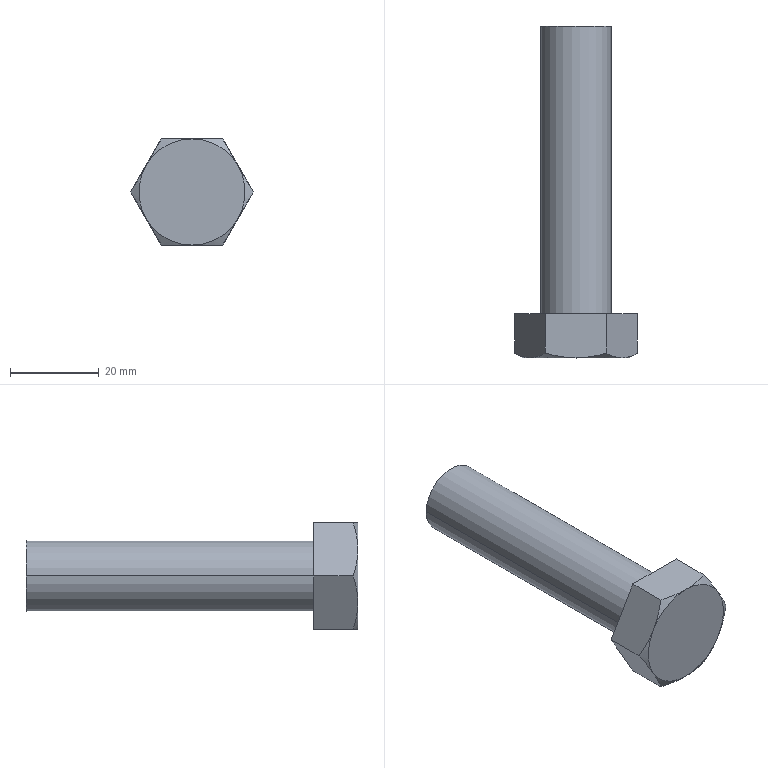Component | SolidWorks | Screw-1 | 1 solid | 17 faces | box 27.71 x 75 x 24 mm | volume 18042 mm3 | plane 9 | cone 6 | cylinder 2 | commonest cylinder face diameters 16 x2
STEP:
#1=COLOUR_RGB('',0.7922,0.8196,0.9333);
#2=FILL_AREA_STYLE_COLOUR('',#1);
#3=FILL_AREA_STYLE('',(#2));
#4=SURFACE_STYLE_FILL_AREA(#3);
#5=SURFACE_SIDE_STYLE('',(#4));
#6=SURFACE_STYLE_USAGE(.BOTH.,#5);
#7=PRESENTATION_STYLE_ASSIGNMENT((#6));
#8=CARTESIAN_POINT('',(-26.588,35.927,34.002));
#9=VERTEX_POINT('',#8);
#10=CARTESIAN_POINT('',(-25.958,35.927,34.002));
#11=VERTEX_POINT('',#10);
#12=CARTESIAN_POINT('',(-26.273,35.927,34.002));
#13=DIRECTION('',(0.,1.,0.));
#14=DIRECTION('',(-1.,0.,0.));
#15=AXIS2_PLACEMENT_3D('',#12,#13,#14);
#16=CIRCLE('',#15,0.315);
#17=EDGE_CURVE('',#9,#11,#16,.T.);
#18=ORIENTED_EDGE('',*,*,#17,.T.);
#19=CARTESIAN_POINT('',(-25.958,38.486,34.002));
#20=VERTEX_POINT('',#19);
#21=CARTESIAN_POINT('',(-25.958,35.927,34.002));
#22=DIRECTION('',(0.,1.,0.));
#23=VECTOR('',#22,39.37);
#24=LINE('',#21,#23);
#25=EDGE_CURVE('',#11,#20,#24,.T.);
#26=ORIENTED_EDGE('',*,*,#25,.T.);
#27=CARTESIAN_POINT('',(-26.588,38.486,34.002));
#28=VERTEX_POINT('',#27);
#29=CARTESIAN_POINT('',(-26.273,38.486,34.002));
#30=DIRECTION('',(0.,1.,0.));
#31=DIRECTION('',(-1.,0.,0.));
#32=AXIS2_PLACEMENT_3D('',#29,#30,#31);
#33=CIRCLE('',#32,0.315);
#34=EDGE_CURVE('',#28,#20,#33,.T.);
#35=ORIENTED_EDGE('',*,*,#34,.F.);
#36=CARTESIAN_POINT('',(-26.588,35.927,34.002));
#37=DIRECTION('',(0.,1.,0.));
#38=VECTOR('',#37,39.37);
#39=LINE('',#36,#38);
#40=EDGE_CURVE('',#9,#28,#39,.T.);
#41=ORIENTED_EDGE('',*,*,#40,.F.);
#42=EDGE_LOOP('',(#18,#26,#35,#41));
#43=FACE_OUTER_BOUND('',#42,.T.);
#44=CARTESIAN_POINT('',(-26.273,35.927,34.002));
#45=DIRECTION('',(0.,1.,0.));
#46=DIRECTION('',(-1.,0.,0.));
#47=AXIS2_PLACEMENT_3D('',#44,#45,#46);
#48=CYLINDRICAL_SURFACE('',#47,0.315);
#49=ADVANCED_FACE('',(#43),#48,.T.);
#50=CARTESIAN_POINT('',(-26.546,35.576,33.53));
#51=VERTEX_POINT('',#50);
#52=CARTESIAN_POINT('',(-26.273,35.533,33.53));
#53=VERTEX_POINT('',#52);
#54=CARTESIAN_POINT('',(-26.546,35.576,33.53));
#55=CARTESIAN_POINT('',(-26.501,35.563,33.53));
#56=CARTESIAN_POINT('',(-26.456,35.552,33.53));
#57=CARTESIAN_POINT('',(-26.365,35.537,33.53));
#58=CARTESIAN_POINT('',(-26.319,35.533,33.53));
#59=CARTESIAN_POINT('',(-26.273,35.533,33.53));
#60=B_SPLINE_CURVE_WITH_KNOTS('',3,(#54,#55,#56,#57,#58,#59),.UNSPECIFIED.,.F.,.F.,(4,2,4),(0.,0.003505,0.007011),.UNSPECIFIED.);
#61=EDGE_CURVE('',#51,#53,#60,.T.);
#62=ORIENTED_EDGE('',*,*,#61,.F.);
#63=CARTESIAN_POINT('',(-26.546,35.927,33.53));
#64=VERTEX_POINT('',#63);
#65=CARTESIAN_POINT('',(-26.546,35.927,33.53));
#66=DIRECTION('',(0.,-1.,0.));
#67=VECTOR('',#66,39.37);
#68=LINE('',#65,#67);
#69=EDGE_CURVE('',#64,#51,#68,.T.);
#70=ORIENTED_EDGE('',*,*,#69,.F.);
#71=CARTESIAN_POINT('',(-26.,35.927,33.53));
#72=VERTEX_POINT('',#71);
#73=CARTESIAN_POINT('',(-26.546,35.927,33.53));
#74=DIRECTION('',(-1.,0.,0.));
#75=VECTOR('',#74,39.37);
#76=LINE('',#73,#75);
#77=EDGE_CURVE('',#72,#64,#76,.T.);
#78=ORIENTED_EDGE('',*,*,#77,.F.);
#79=CARTESIAN_POINT('',(-26.,35.576,33.53));
#80=VERTEX_POINT('',#79);
#81=CARTESIAN_POINT('',(-26.,35.927,33.53));
#82=DIRECTION('',(0.,-1.,0.));
#83=VECTOR('',#82,39.37);
#84=LINE('',#81,#83);
#85=EDGE_CURVE('',#72,#80,#84,.T.);
#86=ORIENTED_EDGE('',*,*,#85,.T.);
#87=CARTESIAN_POINT('',(-26.273,35.533,33.53));
#88=CARTESIAN_POINT('',(-26.226,35.533,33.53));
#89=CARTESIAN_POINT('',(-26.18,35.537,33.53));
#90=CARTESIAN_POINT('',(-26.09,35.552,33.53));
#91=CARTESIAN_POINT('',(-26.045,35.563,33.53));
#92=CARTESIAN_POINT('',(-26.,35.576,33.53));
#93=B_SPLINE_CURVE_WITH_KNOTS('',3,(#87,#88,#89,#90,#91,#92),.UNSPECIFIED.,.F.,.F.,(4,2,4),(0.,0.003505,0.007011),.UNSPECIFIED.);
#94=EDGE_CURVE('',#53,#80,#93,.T.);
#95=ORIENTED_EDGE('',*,*,#94,.F.);
#96=EDGE_LOOP('',(#62,#70,#78,#86,#95));
#97=FACE_OUTER_BOUND('',#96,.T.);
#98=CARTESIAN_POINT('',(-26.,35.533,33.53));
#99=DIRECTION('',(0.,0.,1.));
#100=DIRECTION('',(1.,0.,0.));
#101=AXIS2_PLACEMENT_3D('',#98,#99,#100);
#102=PLANE('',#101);
#103=ADVANCED_FACE('',(#97),#102,.F.);
#104=CARTESIAN_POINT('',(-26.818,35.576,34.002));
#105=VERTEX_POINT('',#104);
#106=CARTESIAN_POINT('',(-26.682,35.533,33.766));
#107=VERTEX_POINT('',#106);
#108=CARTESIAN_POINT('',(-26.818,35.576,34.002));
#109=CARTESIAN_POINT('',(-26.796,35.563,33.964));
#110=CARTESIAN_POINT('',(-26.774,35.552,33.925));
#111=CARTESIAN_POINT('',(-26.728,35.537,33.846));
#112=CARTESIAN_POINT('',(-26.705,35.533,33.807));
#113=CARTESIAN_POINT('',(-26.682,35.533,33.766));
#114=B_SPLINE_CURVE_WITH_KNOTS('',3,(#108,#109,#110,#111,#112,#113),.UNSPECIFIED.,.F.,.F.,(4,2,4),(0.,0.003505,0.007011),.UNSPECIFIED.);
#115=EDGE_CURVE('',#105,#107,#114,.T.);
#116=ORIENTED_EDGE('',*,*,#115,.F.);
#117=CARTESIAN_POINT('',(-26.818,35.927,34.002));
#118=VERTEX_POINT('',#117);
#119=CARTESIAN_POINT('',(-26.818,35.927,34.002));
#120=DIRECTION('',(0.,-1.,0.));
#121=VECTOR('',#120,39.37);
#122=LINE('',#119,#121);
#123=EDGE_CURVE('',#118,#105,#122,.T.);
#124=ORIENTED_EDGE('',*,*,#123,.F.);
#125=CARTESIAN_POINT('',(-26.818,35.927,34.002));
#126=DIRECTION('',(-0.5,0.,0.866));
#127=VECTOR('',#126,39.37);
#128=LINE('',#125,#127);
#129=EDGE_CURVE('',#64,#118,#128,.T.);
#130=ORIENTED_EDGE('',*,*,#129,.F.);
#131=ORIENTED_EDGE('',*,*,#69,.T.);
#132=CARTESIAN_POINT('',(-26.682,35.533,33.766));
#133=CARTESIAN_POINT('',(-26.659,35.533,33.726));
#134=CARTESIAN_POINT('',(-26.636,35.537,33.686));
#135=CARTESIAN_POINT('',(-26.59,35.552,33.608));
#136=CARTESIAN_POINT('',(-26.568,35.563,33.569));
#137=CARTESIAN_POINT('',(-26.546,35.576,33.53));
#138=B_SPLINE_CURVE_WITH_KNOTS('',3,(#132,#133,#134,#135,#136,#137),.UNSPECIFIED.,.F.,.F.,(4,2,4),(0.,0.003505,0.007011),.UNSPECIFIED.);
#139=EDGE_CURVE('',#107,#51,#138,.T.);
#140=ORIENTED_EDGE('',*,*,#139,.F.);
#141=EDGE_LOOP('',(#116,#124,#130,#131,#140));
#142=FACE_OUTER_BOUND('',#141,.T.);
#143=CARTESIAN_POINT('',(-26.546,35.533,33.53));
#144=DIRECTION('',(0.866,0.,0.5));
#145=DIRECTION('',(0.5,0.,-0.866));
#146=AXIS2_PLACEMENT_3D('',#143,#144,#145);
#147=PLANE('',#146);
#148=ADVANCED_FACE('',(#142),#147,.F.);
#149=CARTESIAN_POINT('',(-26.546,35.576,34.475));
#150=VERTEX_POINT('',#149);
#151=CARTESIAN_POINT('',(-26.682,35.533,34.239));
#152=VERTEX_POINT('',#151);
#153=CARTESIAN_POINT('',(-26.546,35.576,34.475));
#154=CARTESIAN_POINT('',(-26.568,35.563,34.436));
#155=CARTESIAN_POINT('',(-26.59,35.552,34.397));
#156=CARTESIAN_POINT('',(-26.636,35.537,34.319));
#157=CARTESIAN_POINT('',(-26.659,35.533,34.279));
#158=CARTESIAN_POINT('',(-26.682,35.533,34.239));
#159=B_SPLINE_CURVE_WITH_KNOTS('',3,(#153,#154,#155,#156,#157,#158),.UNSPECIFIED.,.F.,.F.,(4,2,4),(0.,0.003505,0.007011),.UNSPECIFIED.);
#160=EDGE_CURVE('',#150,#152,#159,.T.);
#161=ORIENTED_EDGE('',*,*,#160,.F.);
#162=CARTESIAN_POINT('',(-26.546,35.927,34.475));
#163=VERTEX_POINT('',#162);
#164=CARTESIAN_POINT('',(-26.546,35.927,34.475));
#165=DIRECTION('',(0.,-1.,0.));
#166=VECTOR('',#165,39.37);
#167=LINE('',#164,#166);
#168=EDGE_CURVE('',#163,#150,#167,.T.);
#169=ORIENTED_EDGE('',*,*,#168,.F.);
#170=CARTESIAN_POINT('',(-26.546,35.927,34.475));
#171=DIRECTION('',(0.5,0.,0.866));
#172=VECTOR('',#171,39.37);
#173=LINE('',#170,#172);
#174=EDGE_CURVE('',#118,#163,#173,.T.);
#175=ORIENTED_EDGE('',*,*,#174,.F.);
#176=ORIENTED_EDGE('',*,*,#123,.T.);
#177=CARTESIAN_POINT('',(-26.682,35.533,34.239));
#178=CARTESIAN_POINT('',(-26.705,35.533,34.198));
#179=CARTESIAN_POINT('',(-26.728,35.537,34.159));
#180=CARTESIAN_POINT('',(-26.774,35.552,34.08));
#181=CARTESIAN_POINT('',(-26.796,35.563,34.041));
#182=CARTESIAN_POINT('',(-26.818,35.576,34.002));
#183=B_SPLINE_CURVE_WITH_KNOTS('',3,(#177,#178,#179,#180,#181,#182),.UNSPECIFIED.,.F.,.F.,(4,2,4),(0.,0.003505,0.007011),.UNSPECIFIED.);
#184=EDGE_CURVE('',#152,#105,#183,.T.);
#185=ORIENTED_EDGE('',*,*,#184,.F.);
#186=EDGE_LOOP('',(#161,#169,#175,#176,#185));
#187=FACE_OUTER_BOUND('',#186,.T.);
#188=CARTESIAN_POINT('',(-26.818,35.533,34.002));
#189=DIRECTION('',(0.866,0.,-0.5));
#190=DIRECTION('',(-0.5,0.,-0.866));
#191=AXIS2_PLACEMENT_3D('',#188,#189,#190);
#192=PLANE('',#191);
#193=ADVANCED_FACE('',(#187),#192,.F.);
#194=CARTESIAN_POINT('',(-26.,35.576,34.475));
#195=VERTEX_POINT('',#194);
#196=CARTESIAN_POINT('',(-26.273,35.533,34.475));
#197=VERTEX_POINT('',#196);
#198=CARTESIAN_POINT('',(-26.,35.576,34.475));
#199=CARTESIAN_POINT('',(-26.045,35.563,34.475));
#200=CARTESIAN_POINT('',(-26.09,35.552,34.475));
#201=CARTESIAN_POINT('',(-26.18,35.537,34.475));
#202=CARTESIAN_POINT('',(-26.226,35.533,34.475));
#203=CARTESIAN_POINT('',(-26.273,35.533,34.475));
#204=B_SPLINE_CURVE_WITH_KNOTS('',3,(#198,#199,#200,#201,#202,#203),.UNSPECIFIED.,.F.,.F.,(4,2,4),(0.,0.003505,0.007011),.UNSPECIFIED.);
#205=EDGE_CURVE('',#195,#197,#204,.T.);
#206=ORIENTED_EDGE('',*,*,#205,.F.);
#207=CARTESIAN_POINT('',(-26.,35.927,34.475));
#208=VERTEX_POINT('',#207);
#209=CARTESIAN_POINT('',(-26.,35.927,34.475));
#210=DIRECTION('',(0.,-1.,0.));
#211=VECTOR('',#210,39.37);
#212=LINE('',#209,#211);
#213=EDGE_CURVE('',#208,#195,#212,.T.);
#214=ORIENTED_EDGE('',*,*,#213,.F.);
#215=CARTESIAN_POINT('',(-26.,35.927,34.475));
#216=DIRECTION('',(1.,0.,0.));
#217=VECTOR('',#216,39.37);
#218=LINE('',#215,#217);
#219=EDGE_CURVE('',#163,#208,#218,.T.);
#220=ORIENTED_EDGE('',*,*,#219,.F.);
#221=ORIENTED_EDGE('',*,*,#168,.T.);
#222=CARTESIAN_POINT('',(-26.273,35.533,34.475));
#223=CARTESIAN_POINT('',(-26.319,35.533,34.475));
#224=CARTESIAN_POINT('',(-26.365,35.537,34.475));
#225=CARTESIAN_POINT('',(-26.456,35.552,34.475));
#226=CARTESIAN_POINT('',(-26.501,35.563,34.475));
#227=CARTESIAN_POINT('',(-26.546,35.576,34.475));
#228=B_SPLINE_CURVE_WITH_KNOTS('',3,(#222,#223,#224,#225,#226,#227),.UNSPECIFIED.,.F.,.F.,(4,2,4),(0.,0.003505,0.007011),.UNSPECIFIED.);
#229=EDGE_CURVE('',#197,#150,#228,.T.);
#230=ORIENTED_EDGE('',*,*,#229,.F.);
#231=EDGE_LOOP('',(#206,#214,#220,#221,#230));
#232=FACE_OUTER_BOUND('',#231,.T.);
#233=CARTESIAN_POINT('',(-26.546,35.533,34.475));
#234=DIRECTION('',(0.,0.,-1.));
#235=DIRECTION('',(-1.,0.,0.));
#236=AXIS2_PLACEMENT_3D('',#233,#234,#235);
#237=PLANE('',#236);
#238=ADVANCED_FACE('',(#232),#237,.F.);
#239=CARTESIAN_POINT('',(-25.727,35.576,34.002));
#240=VERTEX_POINT('',#239);
#241=CARTESIAN_POINT('',(-25.864,35.533,34.239));
#242=VERTEX_POINT('',#241);
#243=CARTESIAN_POINT('',(-25.727,35.576,34.002));
#244=CARTESIAN_POINT('',(-25.75,35.563,34.041));
#245=CARTESIAN_POINT('',(-25.772,35.552,34.08));
#246=CARTESIAN_POINT('',(-25.818,35.537,34.159));
#247=CARTESIAN_POINT('',(-25.841,35.533,34.198));
#248=CARTESIAN_POINT('',(-25.864,35.533,34.239));
#249=B_SPLINE_CURVE_WITH_KNOTS('',3,(#243,#244,#245,#246,#247,#248),.UNSPECIFIED.,.F.,.F.,(4,2,4),(0.,0.003505,0.007011),.UNSPECIFIED.);
#250=EDGE_CURVE('',#240,#242,#249,.T.);
#251=ORIENTED_EDGE('',*,*,#250,.F.);
#252=CARTESIAN_POINT('',(-25.727,35.927,34.002));
#253=VERTEX_POINT('',#252);
#254=CARTESIAN_POINT('',(-25.727,35.927,34.002));
#255=DIRECTION('',(0.,-1.,0.));
#256=VECTOR('',#255,39.37);
#257=LINE('',#254,#256);
#258=EDGE_CURVE('',#253,#240,#257,.T.);
#259=ORIENTED_EDGE('',*,*,#258,.F.);
#260=CARTESIAN_POINT('',(-25.727,35.927,34.002));
#261=DIRECTION('',(0.5,0.,-0.866));
#262=VECTOR('',#261,39.37);
#263=LINE('',#260,#262);
#264=EDGE_CURVE('',#208,#253,#263,.T.);
#265=ORIENTED_EDGE('',*,*,#264,.F.);
#266=ORIENTED_EDGE('',*,*,#213,.T.);
#267=CARTESIAN_POINT('',(-25.864,35.533,34.239));
#268=CARTESIAN_POINT('',(-25.887,35.533,34.279));
#269=CARTESIAN_POINT('',(-25.91,35.537,34.319));
#270=CARTESIAN_POINT('',(-25.955,35.552,34.397));
#271=CARTESIAN_POINT('',(-25.978,35.563,34.436));
#272=CARTESIAN_POINT('',(-26.,35.576,34.475));
#273=B_SPLINE_CURVE_WITH_KNOTS('',3,(#267,#268,#269,#270,#271,#272),.UNSPECIFIED.,.F.,.F.,(4,2,4),(0.,0.003505,0.007011),.UNSPECIFIED.);
#274=EDGE_CURVE('',#242,#195,#273,.T.);
#275=ORIENTED_EDGE('',*,*,#274,.F.);
#276=EDGE_LOOP('',(#251,#259,#265,#266,#275));
#277=FACE_OUTER_BOUND('',#276,.T.);
#278=CARTESIAN_POINT('',(-26.,35.533,34.475));
#279=DIRECTION('',(-0.866,0.,-0.5));
#280=DIRECTION('',(-0.5,0.,0.866));
#281=AXIS2_PLACEMENT_3D('',#278,#279,#280);
#282=PLANE('',#281);
#283=ADVANCED_FACE('',(#277),#282,.F.);
#284=CARTESIAN_POINT('',(-25.864,35.533,33.766));
#285=VERTEX_POINT('',#284);
#286=CARTESIAN_POINT('',(-26.,35.576,33.53));
#287=CARTESIAN_POINT('',(-25.978,35.563,33.569));
#288=CARTESIAN_POINT('',(-25.955,35.552,33.608));
#289=CARTESIAN_POINT('',(-25.91,35.537,33.686));
#290=CARTESIAN_POINT('',(-25.887,35.533,33.726));
#291=CARTESIAN_POINT('',(-25.864,35.533,33.766));
#292=B_SPLINE_CURVE_WITH_KNOTS('',3,(#286,#287,#288,#289,#290,#291),.UNSPECIFIED.,.F.,.F.,(4,2,4),(0.,0.003505,0.007011),.UNSPECIFIED.);
#293=EDGE_CURVE('',#80,#285,#292,.T.);
#294=ORIENTED_EDGE('',*,*,#293,.F.);
#295=ORIENTED_EDGE('',*,*,#85,.F.);
#296=CARTESIAN_POINT('',(-26.,35.927,33.53));
#297=DIRECTION('',(-0.5,0.,-0.866));
#298=VECTOR('',#297,39.37);
#299=LINE('',#296,#298);
#300=EDGE_CURVE('',#253,#72,#299,.T.);
#301=ORIENTED_EDGE('',*,*,#300,.F.);
#302=ORIENTED_EDGE('',*,*,#258,.T.);
#303=CARTESIAN_POINT('',(-25.864,35.533,33.766));
#304=CARTESIAN_POINT('',(-25.841,35.533,33.807));
#305=CARTESIAN_POINT('',(-25.818,35.537,33.846));
#306=CARTESIAN_POINT('',(-25.772,35.552,33.925));
#307=CARTESIAN_POINT('',(-25.75,35.563,33.964));
#308=CARTESIAN_POINT('',(-25.727,35.576,34.002));
#309=B_SPLINE_CURVE_WITH_KNOTS('',3,(#303,#304,#305,#306,#307,#308),.UNSPECIFIED.,.F.,.F.,(4,2,4),(0.,0.003505,0.007011),.UNSPECIFIED.);
#310=EDGE_CURVE('',#285,#240,#309,.T.);
#311=ORIENTED_EDGE('',*,*,#310,.F.);
#312=EDGE_LOOP('',(#294,#295,#301,#302,#311));
#313=FACE_OUTER_BOUND('',#312,.T.);
#314=CARTESIAN_POINT('',(-25.727,35.533,34.002));
#315=DIRECTION('',(-0.866,0.,0.5));
#316=DIRECTION('',(0.5,0.,0.866));
#317=AXIS2_PLACEMENT_3D('',#314,#315,#316);
#318=PLANE('',#317);
#319=ADVANCED_FACE('',(#313),#318,.F.);
#320=CARTESIAN_POINT('',(-26.273,35.533,34.002));
#321=DIRECTION('',(0.,1.,-0.));
#322=DIRECTION('',(0.,0.,1.));
#323=AXIS2_PLACEMENT_3D('',#320,#321,#322);
#324=CIRCLE('',#323,0.4724);
#325=EDGE_CURVE('',#285,#53,#324,.T.);
#326=ORIENTED_EDGE('',*,*,#325,.T.);
#327=ORIENTED_EDGE('',*,*,#94,.T.);
#328=ORIENTED_EDGE('',*,*,#293,.T.);
#329=EDGE_LOOP('',(#326,#327,#328));
#330=FACE_OUTER_BOUND('',#329,.T.);
#331=CARTESIAN_POINT('',(-26.273,35.576,34.002));
#332=DIRECTION('',(0.,1.,-0.));
#333=DIRECTION('',(0.,0.,1.));
#334=AXIS2_PLACEMENT_3D('',#331,#332,#333);
#335=CONICAL_SURFACE('',#334,0.546,1.047);
#336=ADVANCED_FACE('',(#330),#335,.T.);
#337=ORIENTED_EDGE('',*,*,#139,.T.);
#338=ORIENTED_EDGE('',*,*,#61,.T.);
#339=CARTESIAN_POINT('',(-26.273,35.533,34.002));
#340=DIRECTION('',(0.,1.,0.));
#341=DIRECTION('',(-1.,0.,0.));
#342=AXIS2_PLACEMENT_3D('',#339,#340,#341);
#343=CIRCLE('',#342,0.4724);
#344=EDGE_CURVE('',#53,#107,#343,.T.);
#345=ORIENTED_EDGE('',*,*,#344,.T.);
#346=EDGE_LOOP('',(#337,#338,#345));
#347=FACE_OUTER_BOUND('',#346,.T.);
#348=CARTESIAN_POINT('',(-26.273,35.576,34.002));
#349=DIRECTION('',(0.,1.,0.));
#350=DIRECTION('',(-1.,0.,0.));
#351=AXIS2_PLACEMENT_3D('',#348,#349,#350);
#352=CONICAL_SURFACE('',#351,0.546,1.047);
#353=ADVANCED_FACE('',(#347),#352,.T.);
#354=CARTESIAN_POINT('',(-26.273,35.533,34.002));
#355=DIRECTION('',(0.,1.,0.));
#356=DIRECTION('',(0.,0.,1.));
#357=AXIS2_PLACEMENT_3D('',#354,#355,#356);
#358=CIRCLE('',#357,0.4724);
#359=EDGE_CURVE('',#107,#152,#358,.T.);
#360=ORIENTED_EDGE('',*,*,#359,.T.);
#361=ORIENTED_EDGE('',*,*,#184,.T.);
#362=ORIENTED_EDGE('',*,*,#115,.T.);
#363=EDGE_LOOP('',(#360,#361,#362));
#364=FACE_OUTER_BOUND('',#363,.T.);
#365=CARTESIAN_POINT('',(-26.273,35.576,34.002));
#366=DIRECTION('',(0.,1.,0.));
#367=DIRECTION('',(0.,0.,1.));
#368=AXIS2_PLACEMENT_3D('',#365,#366,#367);
#369=CONICAL_SURFACE('',#368,0.546,1.047);
#370=ADVANCED_FACE('',(#364),#369,.T.);
#371=ORIENTED_EDGE('',*,*,#229,.T.);
#372=ORIENTED_EDGE('',*,*,#160,.T.);
#373=CARTESIAN_POINT('',(-26.273,35.533,34.002));
#374=DIRECTION('',(0.,1.,0.));
#375=DIRECTION('',(-1.,0.,0.));
#376=AXIS2_PLACEMENT_3D('',#373,#374,#375);
#377=CIRCLE('',#376,0.4724);
#378=EDGE_CURVE('',#152,#197,#377,.T.);
#379=ORIENTED_EDGE('',*,*,#378,.T.);
#380=EDGE_LOOP('',(#371,#372,#379));
#381=FACE_OUTER_BOUND('',#380,.T.);
#382=CARTESIAN_POINT('',(-26.273,35.576,34.002));
#383=DIRECTION('',(0.,1.,0.));
#384=DIRECTION('',(-1.,0.,0.));
#385=AXIS2_PLACEMENT_3D('',#382,#383,#384);
#386=CONICAL_SURFACE('',#385,0.546,1.047);
#387=ADVANCED_FACE('',(#381),#386,.T.);
#388=CARTESIAN_POINT('',(-26.273,35.533,34.002));
#389=DIRECTION('',(0.,1.,0.));
#390=DIRECTION('',(-1.,0.,0.));
#391=AXIS2_PLACEMENT_3D('',#388,#389,#390);
#392=CIRCLE('',#391,0.4724);
#393=EDGE_CURVE('',#197,#242,#392,.T.);
#394=ORIENTED_EDGE('',*,*,#393,.T.);
#395=ORIENTED_EDGE('',*,*,#274,.T.);
#396=ORIENTED_EDGE('',*,*,#205,.T.);
#397=EDGE_LOOP('',(#394,#395,#396));
#398=FACE_OUTER_BOUND('',#397,.T.);
#399=CARTESIAN_POINT('',(-26.273,35.576,34.002));
#400=DIRECTION('',(0.,1.,0.));
#401=DIRECTION('',(-1.,0.,0.));
#402=AXIS2_PLACEMENT_3D('',#399,#400,#401);
#403=CONICAL_SURFACE('',#402,0.546,1.047);
#404=ADVANCED_FACE('',(#398),#403,.T.);
#405=CARTESIAN_POINT('',(-26.273,35.533,34.002));
#406=DIRECTION('',(0.,1.,0.));
#407=DIRECTION('',(0.,0.,1.));
#408=AXIS2_PLACEMENT_3D('',#405,#406,#407);
#409=CIRCLE('',#408,0.4724);
#410=EDGE_CURVE('',#242,#285,#409,.T.);
#411=ORIENTED_EDGE('',*,*,#410,.T.);
#412=ORIENTED_EDGE('',*,*,#310,.T.);
#413=ORIENTED_EDGE('',*,*,#250,.T.);
#414=EDGE_LOOP('',(#411,#412,#413));
#415=FACE_OUTER_BOUND('',#414,.T.);
#416=CARTESIAN_POINT('',(-26.273,35.576,34.002));
#417=DIRECTION('',(0.,1.,0.));
#418=DIRECTION('',(0.,0.,1.));
#419=AXIS2_PLACEMENT_3D('',#416,#417,#418);
#420=CONICAL_SURFACE('',#419,0.546,1.047);
#421=ADVANCED_FACE('',(#415),#420,.T.);
#422=ORIENTED_EDGE('',*,*,#378,.F.);
#423=ORIENTED_EDGE('',*,*,#359,.F.);
#424=ORIENTED_EDGE('',*,*,#344,.F.);
#425=ORIENTED_EDGE('',*,*,#325,.F.);
#426=ORIENTED_EDGE('',*,*,#410,.F.);
#427=ORIENTED_EDGE('',*,*,#393,.F.);
#428=EDGE_LOOP('',(#422,#423,#424,#425,#426,#427));
#429=FACE_OUTER_BOUND('',#428,.T.);
#430=CARTESIAN_POINT('',(-26.273,35.533,34.002));
#431=DIRECTION('',(0.,-1.,0.));
#432=DIRECTION('',(1.,0.,0.));
#433=AXIS2_PLACEMENT_3D('',#430,#431,#432);
#434=PLANE('',#433);
#435=ADVANCED_FACE('',(#429),#434,.T.);
#436=ORIENTED_EDGE('',*,*,#17,.F.);
#437=CARTESIAN_POINT('',(-26.273,35.927,34.002));
#438=DIRECTION('',(0.,1.,0.));
#439=DIRECTION('',(-1.,0.,0.));
#440=AXIS2_PLACEMENT_3D('',#437,#438,#439);
#441=CIRCLE('',#440,0.315);
#442=EDGE_CURVE('',#11,#9,#441,.T.);
#443=ORIENTED_EDGE('',*,*,#442,.F.);
#444=EDGE_LOOP('',(#436,#443));
#445=FACE_BOUND('',#444,.T.);
#446=ORIENTED_EDGE('',*,*,#174,.T.);
#447=ORIENTED_EDGE('',*,*,#219,.T.);
#448=ORIENTED_EDGE('',*,*,#264,.T.);
#449=ORIENTED_EDGE('',*,*,#300,.T.);
#450=ORIENTED_EDGE('',*,*,#77,.T.);
#451=ORIENTED_EDGE('',*,*,#129,.T.);
#452=EDGE_LOOP('',(#446,#447,#448,#449,#450,#451));
#453=FACE_OUTER_BOUND('',#452,.T.);
#454=CARTESIAN_POINT('',(-36.308,35.927,-26.28));
#455=DIRECTION('',(0.,-1.,0.));
#456=DIRECTION('',(1.,0.,0.));
#457=AXIS2_PLACEMENT_3D('',#454,#455,#456);
#458=PLANE('',#457);
#459=ADVANCED_FACE('',(#445,#453),#458,.F.);
#460=ORIENTED_EDGE('',*,*,#34,.T.);
#461=CARTESIAN_POINT('',(-26.273,38.486,34.002));
#462=DIRECTION('',(0.,1.,0.));
#463=DIRECTION('',(-1.,0.,0.));
#464=AXIS2_PLACEMENT_3D('',#461,#462,#463);
#465=CIRCLE('',#464,0.315);
#466=EDGE_CURVE('',#20,#28,#465,.T.);
#467=ORIENTED_EDGE('',*,*,#466,.T.);
#468=EDGE_LOOP('',(#460,#467));
#469=FACE_OUTER_BOUND('',#468,.T.);
#470=CARTESIAN_POINT('',(-26.273,38.486,34.002));
#471=DIRECTION('',(0.,1.,0.));
#472=DIRECTION('',(-1.,0.,0.));
#473=AXIS2_PLACEMENT_3D('',#470,#471,#472);
#474=PLANE('',#473);
#475=ADVANCED_FACE('',(#469),#474,.T.);
#476=ORIENTED_EDGE('',*,*,#25,.F.);
#477=ORIENTED_EDGE('',*,*,#442,.T.);
#478=ORIENTED_EDGE('',*,*,#40,.T.);
#479=ORIENTED_EDGE('',*,*,#466,.F.);
#480=EDGE_LOOP('',(#476,#477,#478,#479));
#481=FACE_OUTER_BOUND('',#480,.T.);
#482=CARTESIAN_POINT('',(-26.273,35.927,34.002));
#483=DIRECTION('',(0.,1.,0.));
#484=DIRECTION('',(-1.,0.,0.));
#485=AXIS2_PLACEMENT_3D('',#482,#483,#484);
#486=CYLINDRICAL_SURFACE('',#485,0.315);
#487=ADVANCED_FACE('',(#481),#486,.T.);
#488=CLOSED_SHELL('',(#49,#103,#148,#193,#238,#283,#319,#336,#353,#370,#387,#404,#421,#435,#459,#475,#487));
#489=MANIFOLD_SOLID_BREP('',#488);
#490=STYLED_ITEM('',(#7),#489);
#491=(LENGTH_UNIT()NAMED_UNIT(*)SI_UNIT($,.METRE.));
#492=LENGTH_MEASURE_WITH_UNIT(LENGTH_MEASURE(0.0254),#491);
#493=DIMENSIONAL_EXPONENTS(1.,0.,0.,0.,0.,0.,0.);
#494=(CONVERSION_BASED_UNIT('',#492)LENGTH_UNIT()NAMED_UNIT(#493));
#495=UNCERTAINTY_MEASURE_WITH_UNIT(LENGTH_MEASURE(0.00001),#494,'','');
#496=(NAMED_UNIT(*)PLANE_ANGLE_UNIT()SI_UNIT($,.RADIAN.));
#497=(NAMED_UNIT(*)SI_UNIT($,.STERADIAN.)SOLID_ANGLE_UNIT());
#498=(GEOMETRIC_REPRESENTATION_CONTEXT(3)GLOBAL_UNCERTAINTY_ASSIGNED_CONTEXT((#495))GLOBAL_UNIT_ASSIGNED_CONTEXT((#494,#496,#497))REPRESENTATION_CONTEXT('',''));
#499=MECHANICAL_DESIGN_GEOMETRIC_PRESENTATION_REPRESENTATION('',(#490),#498);
#500=PRESENTATION_LAYER_ASSIGNMENT('','',(#490));
#501=CARTESIAN_POINT('',(0.,0.,0.));
#502=DIRECTION('',(0.,0.,1.));
#503=DIRECTION('',(1.,0.,0.));
#504=AXIS2_PLACEMENT_3D('',#501,#502,#503);
#505=(LENGTH_UNIT()NAMED_UNIT(*)SI_UNIT($,.METRE.));
#506=LENGTH_MEASURE_WITH_UNIT(LENGTH_MEASURE(0.0254),#505);
#507=DIMENSIONAL_EXPONENTS(1.,0.,0.,0.,0.,0.,0.);
#508=(CONVERSION_BASED_UNIT('',#506)LENGTH_UNIT()NAMED_UNIT(#507));
#509=UNCERTAINTY_MEASURE_WITH_UNIT(LENGTH_MEASURE(0.00001),#508,'','');
#510=(NAMED_UNIT(*)PLANE_ANGLE_UNIT()SI_UNIT($,.RADIAN.));
#511=(NAMED_UNIT(*)SI_UNIT($,.STERADIAN.)SOLID_ANGLE_UNIT());
#512=(GEOMETRIC_REPRESENTATION_CONTEXT(3)GLOBAL_UNCERTAINTY_ASSIGNED_CONTEXT((#509))GLOBAL_UNIT_ASSIGNED_CONTEXT((#508,#510,#511))REPRESENTATION_CONTEXT('',''));
#513=ADVANCED_BREP_SHAPE_REPRESENTATION('',(#489,#504),#512);